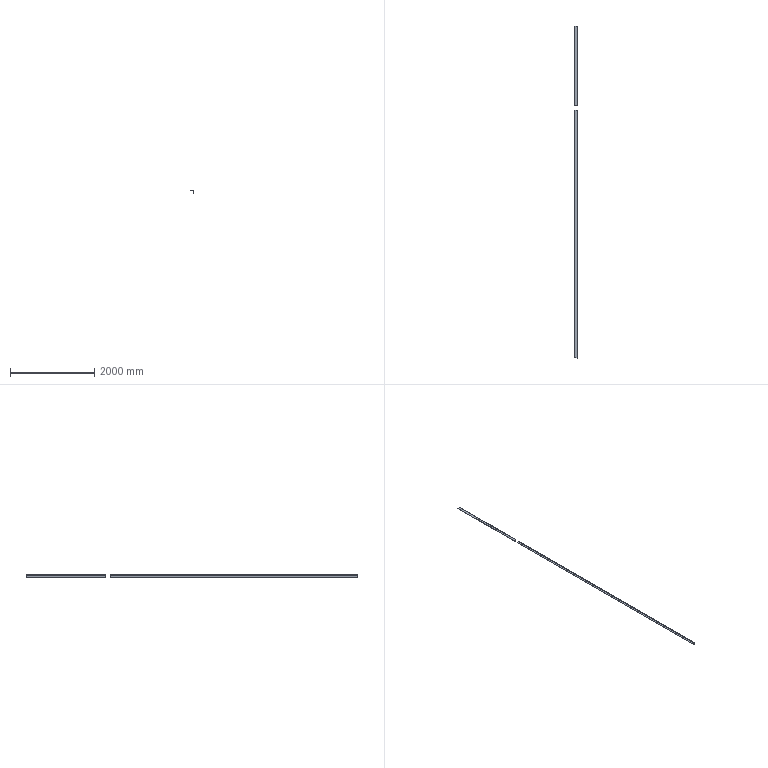Component | SolidWorks | 63#AngleIron-3 | 2 solids | 22 faces | box 63 x 7875 x 63 mm | volume 3857582 mm3 | plane 16 | cylinder 6 | commonest cylinder face diameters 2.667 x4 14 x2
STEP:
#1=COLOUR_RGB('',0.7922,0.8196,0.9333);
#2=FILL_AREA_STYLE_COLOUR('',#1);
#3=FILL_AREA_STYLE('',(#2));
#4=SURFACE_STYLE_FILL_AREA(#3);
#5=SURFACE_SIDE_STYLE('',(#4));
#6=SURFACE_STYLE_USAGE(.BOTH.,#5);
#7=PRESENTATION_STYLE_ASSIGNMENT((#6));
#8=CARTESIAN_POINT('',(81.493,-598.222,187.362));
#9=VERTEX_POINT('',#8);
#10=CARTESIAN_POINT('',(81.493,-598.222,184.882));
#11=VERTEX_POINT('',#10);
#12=CARTESIAN_POINT('',(81.493,-598.222,184.882));
#13=DIRECTION('',(-0.,-0.,-1.));
#14=VECTOR('',#13,39.37);
#15=LINE('',#12,#14);
#16=EDGE_CURVE('',#9,#11,#15,.T.);
#17=ORIENTED_EDGE('',*,*,#16,.T.);
#18=CARTESIAN_POINT('',(81.388,-598.222,184.882));
#19=VERTEX_POINT('',#18);
#20=CARTESIAN_POINT('',(81.493,-598.222,184.882));
#21=DIRECTION('',(-1.,0.,0.));
#22=VECTOR('',#21,39.37);
#23=LINE('',#20,#22);
#24=EDGE_CURVE('',#11,#19,#23,.T.);
#25=ORIENTED_EDGE('',*,*,#24,.T.);
#26=CARTESIAN_POINT('',(81.336,-598.222,184.934));
#27=VERTEX_POINT('',#26);
#28=CARTESIAN_POINT('',(81.388,-598.222,184.934));
#29=DIRECTION('',(0.,1.,-0.));
#30=DIRECTION('',(1.,0.,0.));
#31=AXIS2_PLACEMENT_3D('',#28,#29,#30);
#32=CIRCLE('',#31,0.05249);
#33=EDGE_CURVE('',#19,#27,#32,.T.);
#34=ORIENTED_EDGE('',*,*,#33,.T.);
#35=CARTESIAN_POINT('',(81.336,-598.222,186.929));
#36=VERTEX_POINT('',#35);
#37=CARTESIAN_POINT('',(81.336,-598.222,186.929));
#38=DIRECTION('',(0.,0.,1.));
#39=VECTOR('',#38,39.37);
#40=LINE('',#37,#39);
#41=EDGE_CURVE('',#27,#36,#40,.T.);
#42=ORIENTED_EDGE('',*,*,#41,.T.);
#43=CARTESIAN_POINT('',(81.06,-598.222,187.205));
#44=VERTEX_POINT('',#43);
#45=CARTESIAN_POINT('',(81.06,-598.222,186.929));
#46=DIRECTION('',(-0.,-1.,0.));
#47=DIRECTION('',(-1.,0.,0.));
#48=AXIS2_PLACEMENT_3D('',#45,#46,#47);
#49=CIRCLE('',#48,0.2756);
#50=EDGE_CURVE('',#36,#44,#49,.T.);
#51=ORIENTED_EDGE('',*,*,#50,.T.);
#52=CARTESIAN_POINT('',(79.065,-598.222,187.205));
#53=VERTEX_POINT('',#52);
#54=CARTESIAN_POINT('',(79.065,-598.222,187.205));
#55=DIRECTION('',(-1.,0.,0.));
#56=VECTOR('',#55,39.37);
#57=LINE('',#54,#56);
#58=EDGE_CURVE('',#44,#53,#57,.T.);
#59=ORIENTED_EDGE('',*,*,#58,.T.);
#60=CARTESIAN_POINT('',(79.013,-598.222,187.257));
#61=VERTEX_POINT('',#60);
#62=CARTESIAN_POINT('',(79.065,-598.222,187.257));
#63=DIRECTION('',(0.,1.,-0.));
#64=DIRECTION('',(-1.,0.,0.));
#65=AXIS2_PLACEMENT_3D('',#62,#63,#64);
#66=CIRCLE('',#65,0.05249);
#67=EDGE_CURVE('',#53,#61,#66,.T.);
#68=ORIENTED_EDGE('',*,*,#67,.T.);
#69=CARTESIAN_POINT('',(79.013,-598.222,187.362));
#70=VERTEX_POINT('',#69);
#71=CARTESIAN_POINT('',(79.013,-598.222,187.362));
#72=DIRECTION('',(0.,0.,1.));
#73=VECTOR('',#72,39.37);
#74=LINE('',#71,#73);
#75=EDGE_CURVE('',#61,#70,#74,.T.);
#76=ORIENTED_EDGE('',*,*,#75,.T.);
#77=CARTESIAN_POINT('',(81.493,-598.222,187.362));
#78=DIRECTION('',(1.,-0.,-0.));
#79=VECTOR('',#78,39.37);
#80=LINE('',#77,#79);
#81=EDGE_CURVE('',#70,#9,#80,.T.);
#82=ORIENTED_EDGE('',*,*,#81,.T.);
#83=EDGE_LOOP('',(#17,#25,#34,#42,#51,#59,#68,#76,#82));
#84=FACE_OUTER_BOUND('',#83,.T.);
#85=CARTESIAN_POINT('',(79.065,-598.222,187.257));
#86=DIRECTION('',(-0.,-1.,0.));
#87=DIRECTION('',(-1.,0.,0.));
#88=AXIS2_PLACEMENT_3D('',#85,#86,#87);
#89=PLANE('',#88);
#90=ADVANCED_FACE('',(#84),#89,.F.);
#91=CARTESIAN_POINT('',(79.013,-672.041,187.362));
#92=VERTEX_POINT('',#91);
#93=CARTESIAN_POINT('',(79.013,-598.222,187.362));
#94=DIRECTION('',(-0.,-1.,0.));
#95=VECTOR('',#94,39.37);
#96=LINE('',#93,#95);
#97=EDGE_CURVE('',#70,#92,#96,.T.);
#98=ORIENTED_EDGE('',*,*,#97,.T.);
#99=CARTESIAN_POINT('',(81.493,-672.041,187.362));
#100=VERTEX_POINT('',#99);
#101=CARTESIAN_POINT('',(81.493,-672.041,187.362));
#102=DIRECTION('',(1.,0.,-0.));
#103=VECTOR('',#102,39.37);
#104=LINE('',#101,#103);
#105=EDGE_CURVE('',#92,#100,#104,.T.);
#106=ORIENTED_EDGE('',*,*,#105,.T.);
#107=CARTESIAN_POINT('',(81.493,-598.222,187.362));
#108=DIRECTION('',(-0.,-1.,0.));
#109=VECTOR('',#108,39.37);
#110=LINE('',#107,#109);
#111=EDGE_CURVE('',#9,#100,#110,.T.);
#112=ORIENTED_EDGE('',*,*,#111,.F.);
#113=ORIENTED_EDGE('',*,*,#81,.F.);
#114=EDGE_LOOP('',(#98,#106,#112,#113));
#115=FACE_OUTER_BOUND('',#114,.T.);
#116=CARTESIAN_POINT('',(81.493,-598.222,187.362));
#117=DIRECTION('',(-0.,-0.,-1.));
#118=DIRECTION('',(-1.,0.,0.));
#119=AXIS2_PLACEMENT_3D('',#116,#117,#118);
#120=PLANE('',#119);
#121=ADVANCED_FACE('',(#115),#120,.F.);
#122=CARTESIAN_POINT('',(79.013,-672.041,187.257));
#123=VERTEX_POINT('',#122);
#124=CARTESIAN_POINT('',(79.013,-598.222,187.257));
#125=DIRECTION('',(-0.,-1.,0.));
#126=VECTOR('',#125,39.37);
#127=LINE('',#124,#126);
#128=EDGE_CURVE('',#61,#123,#127,.T.);
#129=ORIENTED_EDGE('',*,*,#128,.T.);
#130=CARTESIAN_POINT('',(79.013,-672.041,187.362));
#131=DIRECTION('',(0.,0.,1.));
#132=VECTOR('',#131,39.37);
#133=LINE('',#130,#132);
#134=EDGE_CURVE('',#123,#92,#133,.T.);
#135=ORIENTED_EDGE('',*,*,#134,.T.);
#136=ORIENTED_EDGE('',*,*,#97,.F.);
#137=ORIENTED_EDGE('',*,*,#75,.F.);
#138=EDGE_LOOP('',(#129,#135,#136,#137));
#139=FACE_OUTER_BOUND('',#138,.T.);
#140=CARTESIAN_POINT('',(79.013,-598.222,187.362));
#141=DIRECTION('',(1.,-0.,-0.));
#142=DIRECTION('',(-0.,-1.,0.));
#143=AXIS2_PLACEMENT_3D('',#140,#141,#142);
#144=PLANE('',#143);
#145=ADVANCED_FACE('',(#139),#144,.F.);
#146=CARTESIAN_POINT('',(79.065,-672.041,187.205));
#147=VERTEX_POINT('',#146);
#148=CARTESIAN_POINT('',(79.065,-598.222,187.205));
#149=DIRECTION('',(-0.,-1.,0.));
#150=VECTOR('',#149,39.37);
#151=LINE('',#148,#150);
#152=EDGE_CURVE('',#53,#147,#151,.T.);
#153=ORIENTED_EDGE('',*,*,#152,.T.);
#154=CARTESIAN_POINT('',(79.065,-672.041,187.257));
#155=DIRECTION('',(0.,1.,0.));
#156=DIRECTION('',(1.,0.,0.));
#157=AXIS2_PLACEMENT_3D('',#154,#155,#156);
#158=CIRCLE('',#157,0.05249);
#159=EDGE_CURVE('',#147,#123,#158,.T.);
#160=ORIENTED_EDGE('',*,*,#159,.T.);
#161=ORIENTED_EDGE('',*,*,#128,.F.);
#162=ORIENTED_EDGE('',*,*,#67,.F.);
#163=EDGE_LOOP('',(#153,#160,#161,#162));
#164=FACE_OUTER_BOUND('',#163,.T.);
#165=CARTESIAN_POINT('',(79.065,-598.222,187.257));
#166=DIRECTION('',(-0.,-1.,0.));
#167=DIRECTION('',(-1.,0.,0.));
#168=AXIS2_PLACEMENT_3D('',#165,#166,#167);
#169=CYLINDRICAL_SURFACE('',#168,0.05249);
#170=ADVANCED_FACE('',(#164),#169,.T.);
#171=CARTESIAN_POINT('',(81.06,-672.041,187.205));
#172=VERTEX_POINT('',#171);
#173=CARTESIAN_POINT('',(81.06,-598.222,187.205));
#174=DIRECTION('',(-0.,-1.,0.));
#175=VECTOR('',#174,39.37);
#176=LINE('',#173,#175);
#177=EDGE_CURVE('',#44,#172,#176,.T.);
#178=ORIENTED_EDGE('',*,*,#177,.T.);
#179=CARTESIAN_POINT('',(79.065,-672.041,187.205));
#180=DIRECTION('',(-1.,0.,0.));
#181=VECTOR('',#180,39.37);
#182=LINE('',#179,#181);
#183=EDGE_CURVE('',#172,#147,#182,.T.);
#184=ORIENTED_EDGE('',*,*,#183,.T.);
#185=ORIENTED_EDGE('',*,*,#152,.F.);
#186=ORIENTED_EDGE('',*,*,#58,.F.);
#187=EDGE_LOOP('',(#178,#184,#185,#186));
#188=FACE_OUTER_BOUND('',#187,.T.);
#189=CARTESIAN_POINT('',(79.065,-598.222,187.205));
#190=DIRECTION('',(0.,0.,1.));
#191=DIRECTION('',(1.,-0.,-0.));
#192=AXIS2_PLACEMENT_3D('',#189,#190,#191);
#193=PLANE('',#192);
#194=ADVANCED_FACE('',(#188),#193,.F.);
#195=CARTESIAN_POINT('',(81.336,-672.041,186.929));
#196=VERTEX_POINT('',#195);
#197=CARTESIAN_POINT('',(81.336,-598.222,186.929));
#198=DIRECTION('',(-0.,-1.,0.));
#199=VECTOR('',#198,39.37);
#200=LINE('',#197,#199);
#201=EDGE_CURVE('',#36,#196,#200,.T.);
#202=ORIENTED_EDGE('',*,*,#201,.T.);
#203=CARTESIAN_POINT('',(81.06,-672.041,186.929));
#204=DIRECTION('',(0.,-1.,-0.));
#205=DIRECTION('',(1.,0.,0.));
#206=AXIS2_PLACEMENT_3D('',#203,#204,#205);
#207=CIRCLE('',#206,0.2756);
#208=EDGE_CURVE('',#196,#172,#207,.T.);
#209=ORIENTED_EDGE('',*,*,#208,.T.);
#210=ORIENTED_EDGE('',*,*,#177,.F.);
#211=ORIENTED_EDGE('',*,*,#50,.F.);
#212=EDGE_LOOP('',(#202,#209,#210,#211));
#213=FACE_OUTER_BOUND('',#212,.T.);
#214=CARTESIAN_POINT('',(81.06,-598.222,186.929));
#215=DIRECTION('',(-0.,-1.,0.));
#216=DIRECTION('',(-1.,0.,0.));
#217=AXIS2_PLACEMENT_3D('',#214,#215,#216);
#218=CYLINDRICAL_SURFACE('',#217,0.2756);
#219=ADVANCED_FACE('',(#213),#218,.F.);
#220=CARTESIAN_POINT('',(81.336,-672.041,184.934));
#221=VERTEX_POINT('',#220);
#222=CARTESIAN_POINT('',(81.336,-598.222,184.934));
#223=DIRECTION('',(-0.,-1.,0.));
#224=VECTOR('',#223,39.37);
#225=LINE('',#222,#224);
#226=EDGE_CURVE('',#27,#221,#225,.T.);
#227=ORIENTED_EDGE('',*,*,#226,.T.);
#228=CARTESIAN_POINT('',(81.336,-672.041,186.929));
#229=DIRECTION('',(0.,0.,1.));
#230=VECTOR('',#229,39.37);
#231=LINE('',#228,#230);
#232=EDGE_CURVE('',#221,#196,#231,.T.);
#233=ORIENTED_EDGE('',*,*,#232,.T.);
#234=ORIENTED_EDGE('',*,*,#201,.F.);
#235=ORIENTED_EDGE('',*,*,#41,.F.);
#236=EDGE_LOOP('',(#227,#233,#234,#235));
#237=FACE_OUTER_BOUND('',#236,.T.);
#238=CARTESIAN_POINT('',(81.336,-598.222,186.929));
#239=DIRECTION('',(1.,-0.,-0.));
#240=DIRECTION('',(-0.,-0.,-1.));
#241=AXIS2_PLACEMENT_3D('',#238,#239,#240);
#242=PLANE('',#241);
#243=ADVANCED_FACE('',(#237),#242,.F.);
#244=CARTESIAN_POINT('',(81.388,-672.041,184.882));
#245=VERTEX_POINT('',#244);
#246=CARTESIAN_POINT('',(81.388,-598.222,184.882));
#247=DIRECTION('',(-0.,-1.,0.));
#248=VECTOR('',#247,39.37);
#249=LINE('',#246,#248);
#250=EDGE_CURVE('',#19,#245,#249,.T.);
#251=ORIENTED_EDGE('',*,*,#250,.T.);
#252=CARTESIAN_POINT('',(81.388,-672.041,184.934));
#253=DIRECTION('',(0.,1.,0.));
#254=DIRECTION('',(1.,0.,0.));
#255=AXIS2_PLACEMENT_3D('',#252,#253,#254);
#256=CIRCLE('',#255,0.05249);
#257=EDGE_CURVE('',#245,#221,#256,.T.);
#258=ORIENTED_EDGE('',*,*,#257,.T.);
#259=ORIENTED_EDGE('',*,*,#226,.F.);
#260=ORIENTED_EDGE('',*,*,#33,.F.);
#261=EDGE_LOOP('',(#251,#258,#259,#260));
#262=FACE_OUTER_BOUND('',#261,.T.);
#263=CARTESIAN_POINT('',(81.388,-598.222,184.934));
#264=DIRECTION('',(-0.,-1.,0.));
#265=DIRECTION('',(-1.,0.,0.));
#266=AXIS2_PLACEMENT_3D('',#263,#264,#265);
#267=CYLINDRICAL_SURFACE('',#266,0.05249);
#268=ADVANCED_FACE('',(#262),#267,.T.);
#269=CARTESIAN_POINT('',(81.493,-672.041,184.882));
#270=VERTEX_POINT('',#269);
#271=CARTESIAN_POINT('',(81.493,-598.222,184.882));
#272=DIRECTION('',(-0.,-1.,0.));
#273=VECTOR('',#272,39.37);
#274=LINE('',#271,#273);
#275=EDGE_CURVE('',#11,#270,#274,.T.);
#276=ORIENTED_EDGE('',*,*,#275,.T.);
#277=CARTESIAN_POINT('',(81.493,-672.041,184.882));
#278=DIRECTION('',(-1.,0.,0.));
#279=VECTOR('',#278,39.37);
#280=LINE('',#277,#279);
#281=EDGE_CURVE('',#270,#245,#280,.T.);
#282=ORIENTED_EDGE('',*,*,#281,.T.);
#283=ORIENTED_EDGE('',*,*,#250,.F.);
#284=ORIENTED_EDGE('',*,*,#24,.F.);
#285=EDGE_LOOP('',(#276,#282,#283,#284));
#286=FACE_OUTER_BOUND('',#285,.T.);
#287=CARTESIAN_POINT('',(81.493,-598.222,184.882));
#288=DIRECTION('',(0.,0.,1.));
#289=DIRECTION('',(1.,-0.,-0.));
#290=AXIS2_PLACEMENT_3D('',#287,#288,#289);
#291=PLANE('',#290);
#292=ADVANCED_FACE('',(#286),#291,.F.);
#293=ORIENTED_EDGE('',*,*,#111,.T.);
#294=CARTESIAN_POINT('',(81.493,-672.041,184.882));
#295=DIRECTION('',(-0.,0.,-1.));
#296=VECTOR('',#295,39.37);
#297=LINE('',#294,#296);
#298=EDGE_CURVE('',#100,#270,#297,.T.);
#299=ORIENTED_EDGE('',*,*,#298,.T.);
#300=ORIENTED_EDGE('',*,*,#275,.F.);
#301=ORIENTED_EDGE('',*,*,#16,.F.);
#302=EDGE_LOOP('',(#293,#299,#300,#301));
#303=FACE_OUTER_BOUND('',#302,.T.);
#304=CARTESIAN_POINT('',(81.493,-598.222,184.882));
#305=DIRECTION('',(-1.,0.,0.));
#306=DIRECTION('',(0.,1.,-0.));
#307=AXIS2_PLACEMENT_3D('',#304,#305,#306);
#308=PLANE('',#307);
#309=ADVANCED_FACE('',(#303),#308,.F.);
#310=ORIENTED_EDGE('',*,*,#105,.F.);
#311=ORIENTED_EDGE('',*,*,#134,.F.);
#312=ORIENTED_EDGE('',*,*,#159,.F.);
#313=ORIENTED_EDGE('',*,*,#183,.F.);
#314=ORIENTED_EDGE('',*,*,#208,.F.);
#315=ORIENTED_EDGE('',*,*,#232,.F.);
#316=ORIENTED_EDGE('',*,*,#257,.F.);
#317=ORIENTED_EDGE('',*,*,#281,.F.);
#318=ORIENTED_EDGE('',*,*,#298,.F.);
#319=EDGE_LOOP('',(#310,#311,#312,#313,#314,#315,#316,#317,#318));
#320=FACE_OUTER_BOUND('',#319,.T.);
#321=CARTESIAN_POINT('',(-68.113,-672.041,23.622));
#322=DIRECTION('',(0.,1.,-0.));
#323=DIRECTION('',(0.,0.,1.));
#324=AXIS2_PLACEMENT_3D('',#321,#322,#323);
#325=PLANE('',#324);
#326=ADVANCED_FACE('',(#320),#325,.F.);
#327=CLOSED_SHELL('',(#90,#121,#145,#170,#194,#219,#243,#268,#292,#309,#326));
#328=MANIFOLD_SOLID_BREP('',#327);
#329=STYLED_ITEM('',(#7),#328);
#330=PRESENTATION_LAYER_ASSIGNMENT('','',(#329));
#331=(LENGTH_UNIT()NAMED_UNIT(*)SI_UNIT($,.METRE.));
#332=LENGTH_MEASURE_WITH_UNIT(LENGTH_MEASURE(0.0254),#331);
#333=DIMENSIONAL_EXPONENTS(1.,0.,0.,0.,0.,0.,0.);
#334=(CONVERSION_BASED_UNIT('',#332)LENGTH_UNIT()NAMED_UNIT(#333));
#335=UNCERTAINTY_MEASURE_WITH_UNIT(LENGTH_MEASURE(0.00001),#334,'','');
#336=(NAMED_UNIT(*)PLANE_ANGLE_UNIT()SI_UNIT($,.RADIAN.));
#337=(NAMED_UNIT(*)SI_UNIT($,.STERADIAN.)SOLID_ANGLE_UNIT());
#338=(GEOMETRIC_REPRESENTATION_CONTEXT(3)GLOBAL_UNCERTAINTY_ASSIGNED_CONTEXT((#335))GLOBAL_UNIT_ASSIGNED_CONTEXT((#334,#336,#337))REPRESENTATION_CONTEXT('',''));
#339=MECHANICAL_DESIGN_GEOMETRIC_PRESENTATION_REPRESENTATION('',(#329),#338);
#340=CARTESIAN_POINT('',(81.493,-676.962,187.362));
#341=VERTEX_POINT('',#340);
#342=CARTESIAN_POINT('',(81.493,-908.262,187.362));
#343=VERTEX_POINT('',#342);
#344=CARTESIAN_POINT('',(81.493,-598.222,187.362));
#345=DIRECTION('',(-0.,-1.,0.));
#346=VECTOR('',#345,39.37);
#347=LINE('',#344,#346);
#348=EDGE_CURVE('',#341,#343,#347,.T.);
#349=ORIENTED_EDGE('',*,*,#348,.T.);
#350=CARTESIAN_POINT('',(81.493,-908.262,184.882));
#351=VERTEX_POINT('',#350);
#352=CARTESIAN_POINT('',(81.493,-908.262,184.882));
#353=DIRECTION('',(-0.,0.,-1.));
#354=VECTOR('',#353,39.37);
#355=LINE('',#352,#354);
#356=EDGE_CURVE('',#343,#351,#355,.T.);
#357=ORIENTED_EDGE('',*,*,#356,.T.);
#358=CARTESIAN_POINT('',(81.493,-676.962,184.882));
#359=VERTEX_POINT('',#358);
#360=CARTESIAN_POINT('',(81.493,-598.222,184.882));
#361=DIRECTION('',(-0.,-1.,0.));
#362=VECTOR('',#361,39.37);
#363=LINE('',#360,#362);
#364=EDGE_CURVE('',#359,#351,#363,.T.);
#365=ORIENTED_EDGE('',*,*,#364,.F.);
#366=CARTESIAN_POINT('',(81.493,-676.962,184.882));
#367=DIRECTION('',(0.,0.,1.));
#368=VECTOR('',#367,39.37);
#369=LINE('',#366,#368);
#370=EDGE_CURVE('',#359,#341,#369,.T.);
#371=ORIENTED_EDGE('',*,*,#370,.T.);
#372=EDGE_LOOP('',(#349,#357,#365,#371));
#373=FACE_OUTER_BOUND('',#372,.T.);
#374=CARTESIAN_POINT('',(81.493,-598.222,184.882));
#375=DIRECTION('',(-1.,0.,0.));
#376=DIRECTION('',(0.,1.,-0.));
#377=AXIS2_PLACEMENT_3D('',#374,#375,#376);
#378=PLANE('',#377);
#379=ADVANCED_FACE('',(#373),#378,.F.);
#380=ORIENTED_EDGE('',*,*,#364,.T.);
#381=CARTESIAN_POINT('',(81.388,-908.262,184.882));
#382=VERTEX_POINT('',#381);
#383=CARTESIAN_POINT('',(81.493,-908.262,184.882));
#384=DIRECTION('',(-1.,0.,0.));
#385=VECTOR('',#384,39.37);
#386=LINE('',#383,#385);
#387=EDGE_CURVE('',#351,#382,#386,.T.);
#388=ORIENTED_EDGE('',*,*,#387,.T.);
#389=CARTESIAN_POINT('',(81.388,-676.962,184.882));
#390=VERTEX_POINT('',#389);
#391=CARTESIAN_POINT('',(81.388,-598.222,184.882));
#392=DIRECTION('',(-0.,-1.,0.));
#393=VECTOR('',#392,39.37);
#394=LINE('',#391,#393);
#395=EDGE_CURVE('',#390,#382,#394,.T.);
#396=ORIENTED_EDGE('',*,*,#395,.F.);
#397=CARTESIAN_POINT('',(81.493,-676.962,184.882));
#398=DIRECTION('',(1.,0.,-0.));
#399=VECTOR('',#398,39.37);
#400=LINE('',#397,#399);
#401=EDGE_CURVE('',#390,#359,#400,.T.);
#402=ORIENTED_EDGE('',*,*,#401,.T.);
#403=EDGE_LOOP('',(#380,#388,#396,#402));
#404=FACE_OUTER_BOUND('',#403,.T.);
#405=CARTESIAN_POINT('',(81.493,-598.222,184.882));
#406=DIRECTION('',(0.,0.,1.));
#407=DIRECTION('',(1.,-0.,-0.));
#408=AXIS2_PLACEMENT_3D('',#405,#406,#407);
#409=PLANE('',#408);
#410=ADVANCED_FACE('',(#404),#409,.F.);
#411=ORIENTED_EDGE('',*,*,#395,.T.);
#412=CARTESIAN_POINT('',(81.336,-908.262,184.934));
#413=VERTEX_POINT('',#412);
#414=CARTESIAN_POINT('',(81.388,-908.262,184.934));
#415=DIRECTION('',(0.,1.,0.));
#416=DIRECTION('',(1.,0.,0.));
#417=AXIS2_PLACEMENT_3D('',#414,#415,#416);
#418=CIRCLE('',#417,0.05249);
#419=EDGE_CURVE('',#382,#413,#418,.T.);
#420=ORIENTED_EDGE('',*,*,#419,.T.);
#421=CARTESIAN_POINT('',(81.336,-676.962,184.934));
#422=VERTEX_POINT('',#421);
#423=CARTESIAN_POINT('',(81.336,-598.222,184.934));
#424=DIRECTION('',(-0.,-1.,0.));
#425=VECTOR('',#424,39.37);
#426=LINE('',#423,#425);
#427=EDGE_CURVE('',#422,#413,#426,.T.);
#428=ORIENTED_EDGE('',*,*,#427,.F.);
#429=CARTESIAN_POINT('',(81.388,-676.962,184.934));
#430=DIRECTION('',(0.,-1.,-0.));
#431=DIRECTION('',(-1.,0.,0.));
#432=AXIS2_PLACEMENT_3D('',#429,#430,#431);
#433=CIRCLE('',#432,0.05249);
#434=EDGE_CURVE('',#422,#390,#433,.T.);
#435=ORIENTED_EDGE('',*,*,#434,.T.);
#436=EDGE_LOOP('',(#411,#420,#428,#435));
#437=FACE_OUTER_BOUND('',#436,.T.);
#438=CARTESIAN_POINT('',(81.388,-598.222,184.934));
#439=DIRECTION('',(-0.,-1.,0.));
#440=DIRECTION('',(-1.,0.,0.));
#441=AXIS2_PLACEMENT_3D('',#438,#439,#440);
#442=CYLINDRICAL_SURFACE('',#441,0.05249);
#443=ADVANCED_FACE('',(#437),#442,.T.);
#444=ORIENTED_EDGE('',*,*,#427,.T.);
#445=CARTESIAN_POINT('',(81.336,-908.262,186.929));
#446=VERTEX_POINT('',#445);
#447=CARTESIAN_POINT('',(81.336,-908.262,186.929));
#448=DIRECTION('',(0.,0.,1.));
#449=VECTOR('',#448,39.37);
#450=LINE('',#447,#449);
#451=EDGE_CURVE('',#413,#446,#450,.T.);
#452=ORIENTED_EDGE('',*,*,#451,.T.);
#453=CARTESIAN_POINT('',(81.336,-676.962,186.929));
#454=VERTEX_POINT('',#453);
#455=CARTESIAN_POINT('',(81.336,-598.222,186.929));
#456=DIRECTION('',(-0.,-1.,0.));
#457=VECTOR('',#456,39.37);
#458=LINE('',#455,#457);
#459=EDGE_CURVE('',#454,#446,#458,.T.);
#460=ORIENTED_EDGE('',*,*,#459,.F.);
#461=CARTESIAN_POINT('',(81.336,-676.962,186.929));
#462=DIRECTION('',(-0.,-0.,-1.));
#463=VECTOR('',#462,39.37);
#464=LINE('',#461,#463);
#465=EDGE_CURVE('',#454,#422,#464,.T.);
#466=ORIENTED_EDGE('',*,*,#465,.T.);
#467=EDGE_LOOP('',(#444,#452,#460,#466));
#468=FACE_OUTER_BOUND('',#467,.T.);
#469=CARTESIAN_POINT('',(81.336,-598.222,186.929));
#470=DIRECTION('',(1.,-0.,-0.));
#471=DIRECTION('',(-0.,-0.,-1.));
#472=AXIS2_PLACEMENT_3D('',#469,#470,#471);
#473=PLANE('',#472);
#474=ADVANCED_FACE('',(#468),#473,.F.);
#475=ORIENTED_EDGE('',*,*,#459,.T.);
#476=CARTESIAN_POINT('',(81.06,-908.262,187.205));
#477=VERTEX_POINT('',#476);
#478=CARTESIAN_POINT('',(81.06,-908.262,186.929));
#479=DIRECTION('',(0.,-1.,-0.));
#480=DIRECTION('',(1.,0.,0.));
#481=AXIS2_PLACEMENT_3D('',#478,#479,#480);
#482=CIRCLE('',#481,0.2756);
#483=EDGE_CURVE('',#446,#477,#482,.T.);
#484=ORIENTED_EDGE('',*,*,#483,.T.);
#485=CARTESIAN_POINT('',(81.06,-676.962,187.205));
#486=VERTEX_POINT('',#485);
#487=CARTESIAN_POINT('',(81.06,-598.222,187.205));
#488=DIRECTION('',(-0.,-1.,0.));
#489=VECTOR('',#488,39.37);
#490=LINE('',#487,#489);
#491=EDGE_CURVE('',#486,#477,#490,.T.);
#492=ORIENTED_EDGE('',*,*,#491,.F.);
#493=CARTESIAN_POINT('',(81.06,-676.962,186.929));
#494=DIRECTION('',(0.,1.,0.));
#495=DIRECTION('',(-1.,0.,0.));
#496=AXIS2_PLACEMENT_3D('',#493,#494,#495);
#497=CIRCLE('',#496,0.2756);
#498=EDGE_CURVE('',#486,#454,#497,.T.);
#499=ORIENTED_EDGE('',*,*,#498,.T.);
#500=EDGE_LOOP('',(#475,#484,#492,#499));
#501=FACE_OUTER_BOUND('',#500,.T.);
#502=CARTESIAN_POINT('',(81.06,-598.222,186.929));
#503=DIRECTION('',(-0.,-1.,0.));
#504=DIRECTION('',(-1.,0.,0.));
#505=AXIS2_PLACEMENT_3D('',#502,#503,#504);
#506=CYLINDRICAL_SURFACE('',#505,0.2756);
#507=ADVANCED_FACE('',(#501),#506,.F.);
#508=ORIENTED_EDGE('',*,*,#491,.T.);
#509=CARTESIAN_POINT('',(79.065,-908.262,187.205));
#510=VERTEX_POINT('',#509);
#511=CARTESIAN_POINT('',(79.065,-908.262,187.205));
#512=DIRECTION('',(-1.,0.,0.));
#513=VECTOR('',#512,39.37);
#514=LINE('',#511,#513);
#515=EDGE_CURVE('',#477,#510,#514,.T.);
#516=ORIENTED_EDGE('',*,*,#515,.T.);
#517=CARTESIAN_POINT('',(79.065,-676.962,187.205));
#518=VERTEX_POINT('',#517);
#519=CARTESIAN_POINT('',(79.065,-598.222,187.205));
#520=DIRECTION('',(-0.,-1.,0.));
#521=VECTOR('',#520,39.37);
#522=LINE('',#519,#521);
#523=EDGE_CURVE('',#518,#510,#522,.T.);
#524=ORIENTED_EDGE('',*,*,#523,.F.);
#525=CARTESIAN_POINT('',(79.065,-676.962,187.205));
#526=DIRECTION('',(1.,0.,-0.));
#527=VECTOR('',#526,39.37);
#528=LINE('',#525,#527);
#529=EDGE_CURVE('',#518,#486,#528,.T.);
#530=ORIENTED_EDGE('',*,*,#529,.T.);
#531=EDGE_LOOP('',(#508,#516,#524,#530));
#532=FACE_OUTER_BOUND('',#531,.T.);
#533=CARTESIAN_POINT('',(79.065,-598.222,187.205));
#534=DIRECTION('',(0.,0.,1.));
#535=DIRECTION('',(1.,-0.,-0.));
#536=AXIS2_PLACEMENT_3D('',#533,#534,#535);
#537=PLANE('',#536);
#538=ADVANCED_FACE('',(#532),#537,.F.);
#539=ORIENTED_EDGE('',*,*,#523,.T.);
#540=CARTESIAN_POINT('',(79.013,-908.262,187.257));
#541=VERTEX_POINT('',#540);
#542=CARTESIAN_POINT('',(79.065,-908.262,187.257));
#543=DIRECTION('',(0.,1.,0.));
#544=DIRECTION('',(1.,0.,0.));
#545=AXIS2_PLACEMENT_3D('',#542,#543,#544);
#546=CIRCLE('',#545,0.05249);
#547=EDGE_CURVE('',#510,#541,#546,.T.);
#548=ORIENTED_EDGE('',*,*,#547,.T.);
#549=CARTESIAN_POINT('',(79.013,-676.962,187.257));
#550=VERTEX_POINT('',#549);
#551=CARTESIAN_POINT('',(79.013,-598.222,187.257));
#552=DIRECTION('',(-0.,-1.,0.));
#553=VECTOR('',#552,39.37);
#554=LINE('',#551,#553);
#555=EDGE_CURVE('',#550,#541,#554,.T.);
#556=ORIENTED_EDGE('',*,*,#555,.F.);
#557=CARTESIAN_POINT('',(79.065,-676.962,187.257));
#558=DIRECTION('',(0.,-1.,-0.));
#559=DIRECTION('',(-1.,0.,0.));
#560=AXIS2_PLACEMENT_3D('',#557,#558,#559);
#561=CIRCLE('',#560,0.05249);
#562=EDGE_CURVE('',#550,#518,#561,.T.);
#563=ORIENTED_EDGE('',*,*,#562,.T.);
#564=EDGE_LOOP('',(#539,#548,#556,#563));
#565=FACE_OUTER_BOUND('',#564,.T.);
#566=CARTESIAN_POINT('',(79.065,-598.222,187.257));
#567=DIRECTION('',(-0.,-1.,0.));
#568=DIRECTION('',(-1.,0.,0.));
#569=AXIS2_PLACEMENT_3D('',#566,#567,#568);
#570=CYLINDRICAL_SURFACE('',#569,0.05249);
#571=ADVANCED_FACE('',(#565),#570,.T.);
#572=ORIENTED_EDGE('',*,*,#555,.T.);
#573=CARTESIAN_POINT('',(79.013,-908.262,187.362));
#574=VERTEX_POINT('',#573);
#575=CARTESIAN_POINT('',(79.013,-908.262,187.362));
#576=DIRECTION('',(0.,0.,1.));
#577=VECTOR('',#576,39.37);
#578=LINE('',#575,#577);
#579=EDGE_CURVE('',#541,#574,#578,.T.);
#580=ORIENTED_EDGE('',*,*,#579,.T.);
#581=CARTESIAN_POINT('',(79.013,-676.962,187.362));
#582=VERTEX_POINT('',#581);
#583=CARTESIAN_POINT('',(79.013,-598.222,187.362));
#584=DIRECTION('',(-0.,-1.,0.));
#585=VECTOR('',#584,39.37);
#586=LINE('',#583,#585);
#587=EDGE_CURVE('',#582,#574,#586,.T.);
#588=ORIENTED_EDGE('',*,*,#587,.F.);
#589=CARTESIAN_POINT('',(79.013,-676.962,187.362));
#590=DIRECTION('',(-0.,0.,-1.));
#591=VECTOR('',#590,39.37);
#592=LINE('',#589,#591);
#593=EDGE_CURVE('',#582,#550,#592,.T.);
#594=ORIENTED_EDGE('',*,*,#593,.T.);
#595=EDGE_LOOP('',(#572,#580,#588,#594));
#596=FACE_OUTER_BOUND('',#595,.T.);
#597=CARTESIAN_POINT('',(79.013,-598.222,187.362));
#598=DIRECTION('',(1.,-0.,-0.));
#599=DIRECTION('',(-0.,-1.,0.));
#600=AXIS2_PLACEMENT_3D('',#597,#598,#599);
#601=PLANE('',#600);
#602=ADVANCED_FACE('',(#596),#601,.F.);
#603=ORIENTED_EDGE('',*,*,#587,.T.);
#604=CARTESIAN_POINT('',(81.493,-908.262,187.362));
#605=DIRECTION('',(1.,0.,-0.));
#606=VECTOR('',#605,39.37);
#607=LINE('',#604,#606);
#608=EDGE_CURVE('',#574,#343,#607,.T.);
#609=ORIENTED_EDGE('',*,*,#608,.T.);
#610=ORIENTED_EDGE('',*,*,#348,.F.);
#611=CARTESIAN_POINT('',(81.493,-676.962,187.362));
#612=DIRECTION('',(-1.,0.,0.));
#613=VECTOR('',#612,39.37);
#614=LINE('',#611,#613);
#615=EDGE_CURVE('',#341,#582,#614,.T.);
#616=ORIENTED_EDGE('',*,*,#615,.T.);
#617=EDGE_LOOP('',(#603,#609,#610,#616));
#618=FACE_OUTER_BOUND('',#617,.T.);
#619=CARTESIAN_POINT('',(81.493,-598.222,187.362));
#620=DIRECTION('',(-0.,-0.,-1.));
#621=DIRECTION('',(-1.,0.,0.));
#622=AXIS2_PLACEMENT_3D('',#619,#620,#621);
#623=PLANE('',#622);
#624=ADVANCED_FACE('',(#618),#623,.F.);
#625=ORIENTED_EDGE('',*,*,#401,.F.);
#626=ORIENTED_EDGE('',*,*,#434,.F.);
#627=ORIENTED_EDGE('',*,*,#465,.F.);
#628=ORIENTED_EDGE('',*,*,#498,.F.);
#629=ORIENTED_EDGE('',*,*,#529,.F.);
#630=ORIENTED_EDGE('',*,*,#562,.F.);
#631=ORIENTED_EDGE('',*,*,#593,.F.);
#632=ORIENTED_EDGE('',*,*,#615,.F.);
#633=ORIENTED_EDGE('',*,*,#370,.F.);
#634=EDGE_LOOP('',(#625,#626,#627,#628,#629,#630,#631,#632,#633));
#635=FACE_OUTER_BOUND('',#634,.T.);
#636=CARTESIAN_POINT('',(-68.113,-676.962,23.622));
#637=DIRECTION('',(0.,-1.,0.));
#638=DIRECTION('',(0.,-0.,-1.));
#639=AXIS2_PLACEMENT_3D('',#636,#637,#638);
#640=PLANE('',#639);
#641=ADVANCED_FACE('',(#635),#640,.F.);
#642=ORIENTED_EDGE('',*,*,#608,.F.);
#643=ORIENTED_EDGE('',*,*,#579,.F.);
#644=ORIENTED_EDGE('',*,*,#547,.F.);
#645=ORIENTED_EDGE('',*,*,#515,.F.);
#646=ORIENTED_EDGE('',*,*,#483,.F.);
#647=ORIENTED_EDGE('',*,*,#451,.F.);
#648=ORIENTED_EDGE('',*,*,#419,.F.);
#649=ORIENTED_EDGE('',*,*,#387,.F.);
#650=ORIENTED_EDGE('',*,*,#356,.F.);
#651=EDGE_LOOP('',(#642,#643,#644,#645,#646,#647,#648,#649,#650));
#652=FACE_OUTER_BOUND('',#651,.T.);
#653=CARTESIAN_POINT('',(-68.113,-908.262,23.622));
#654=DIRECTION('',(0.,1.,-0.));
#655=DIRECTION('',(0.,0.,1.));
#656=AXIS2_PLACEMENT_3D('',#653,#654,#655);
#657=PLANE('',#656);
#658=ADVANCED_FACE('',(#652),#657,.F.);
#659=CLOSED_SHELL('',(#379,#410,#443,#474,#507,#538,#571,#602,#624,#641,#658));
#660=MANIFOLD_SOLID_BREP('',#659);
#661=CARTESIAN_POINT('',(0.,0.,0.));
#662=DIRECTION('',(0.,0.,1.));
#663=DIRECTION('',(1.,0.,0.));
#664=AXIS2_PLACEMENT_3D('',#661,#662,#663);
#665=(LENGTH_UNIT()NAMED_UNIT(*)SI_UNIT($,.METRE.));
#666=LENGTH_MEASURE_WITH_UNIT(LENGTH_MEASURE(0.0254),#665);
#667=DIMENSIONAL_EXPONENTS(1.,0.,0.,0.,0.,0.,0.);
#668=(CONVERSION_BASED_UNIT('',#666)LENGTH_UNIT()NAMED_UNIT(#667));
#669=UNCERTAINTY_MEASURE_WITH_UNIT(LENGTH_MEASURE(0.00001),#668,'','');
#670=(NAMED_UNIT(*)PLANE_ANGLE_UNIT()SI_UNIT($,.RADIAN.));
#671=(NAMED_UNIT(*)SI_UNIT($,.STERADIAN.)SOLID_ANGLE_UNIT());
#672=(GEOMETRIC_REPRESENTATION_CONTEXT(3)GLOBAL_UNCERTAINTY_ASSIGNED_CONTEXT((#669))GLOBAL_UNIT_ASSIGNED_CONTEXT((#668,#670,#671))REPRESENTATION_CONTEXT('',''));
#673=ADVANCED_BREP_SHAPE_REPRESENTATION('',(#660,#328,#664),#672);
#674=COLOUR_RGB('',0.7922,0.8196,0.9333);
#675=FILL_AREA_STYLE_COLOUR('',#674);
#676=FILL_AREA_STYLE('',(#675));
#677=SURFACE_STYLE_FILL_AREA(#676);
#678=SURFACE_SIDE_STYLE('',(#677));
#679=SURFACE_STYLE_USAGE(.BOTH.,#678);
#680=PRESENTATION_STYLE_ASSIGNMENT((#679));
#681=STYLED_ITEM('',(#680),#660);
#682=(LENGTH_UNIT()NAMED_UNIT(*)SI_UNIT($,.METRE.));
#683=LENGTH_MEASURE_WITH_UNIT(LENGTH_MEASURE(0.0254),#682);
#684=DIMENSIONAL_EXPONENTS(1.,0.,0.,0.,0.,0.,0.);
#685=(CONVERSION_BASED_UNIT('',#683)LENGTH_UNIT()NAMED_UNIT(#684));
#686=UNCERTAINTY_MEASURE_WITH_UNIT(LENGTH_MEASURE(0.00001),#685,'','');
#687=(NAMED_UNIT(*)PLANE_ANGLE_UNIT()SI_UNIT($,.RADIAN.));
#688=(NAMED_UNIT(*)SI_UNIT($,.STERADIAN.)SOLID_ANGLE_UNIT());
#689=(GEOMETRIC_REPRESENTATION_CONTEXT(3)GLOBAL_UNCERTAINTY_ASSIGNED_CONTEXT((#686))GLOBAL_UNIT_ASSIGNED_CONTEXT((#685,#687,#688))REPRESENTATION_CONTEXT('',''));
#690=MECHANICAL_DESIGN_GEOMETRIC_PRESENTATION_REPRESENTATION('',(#681),#689);
#691=PRESENTATION_LAYER_ASSIGNMENT('','',(#681));